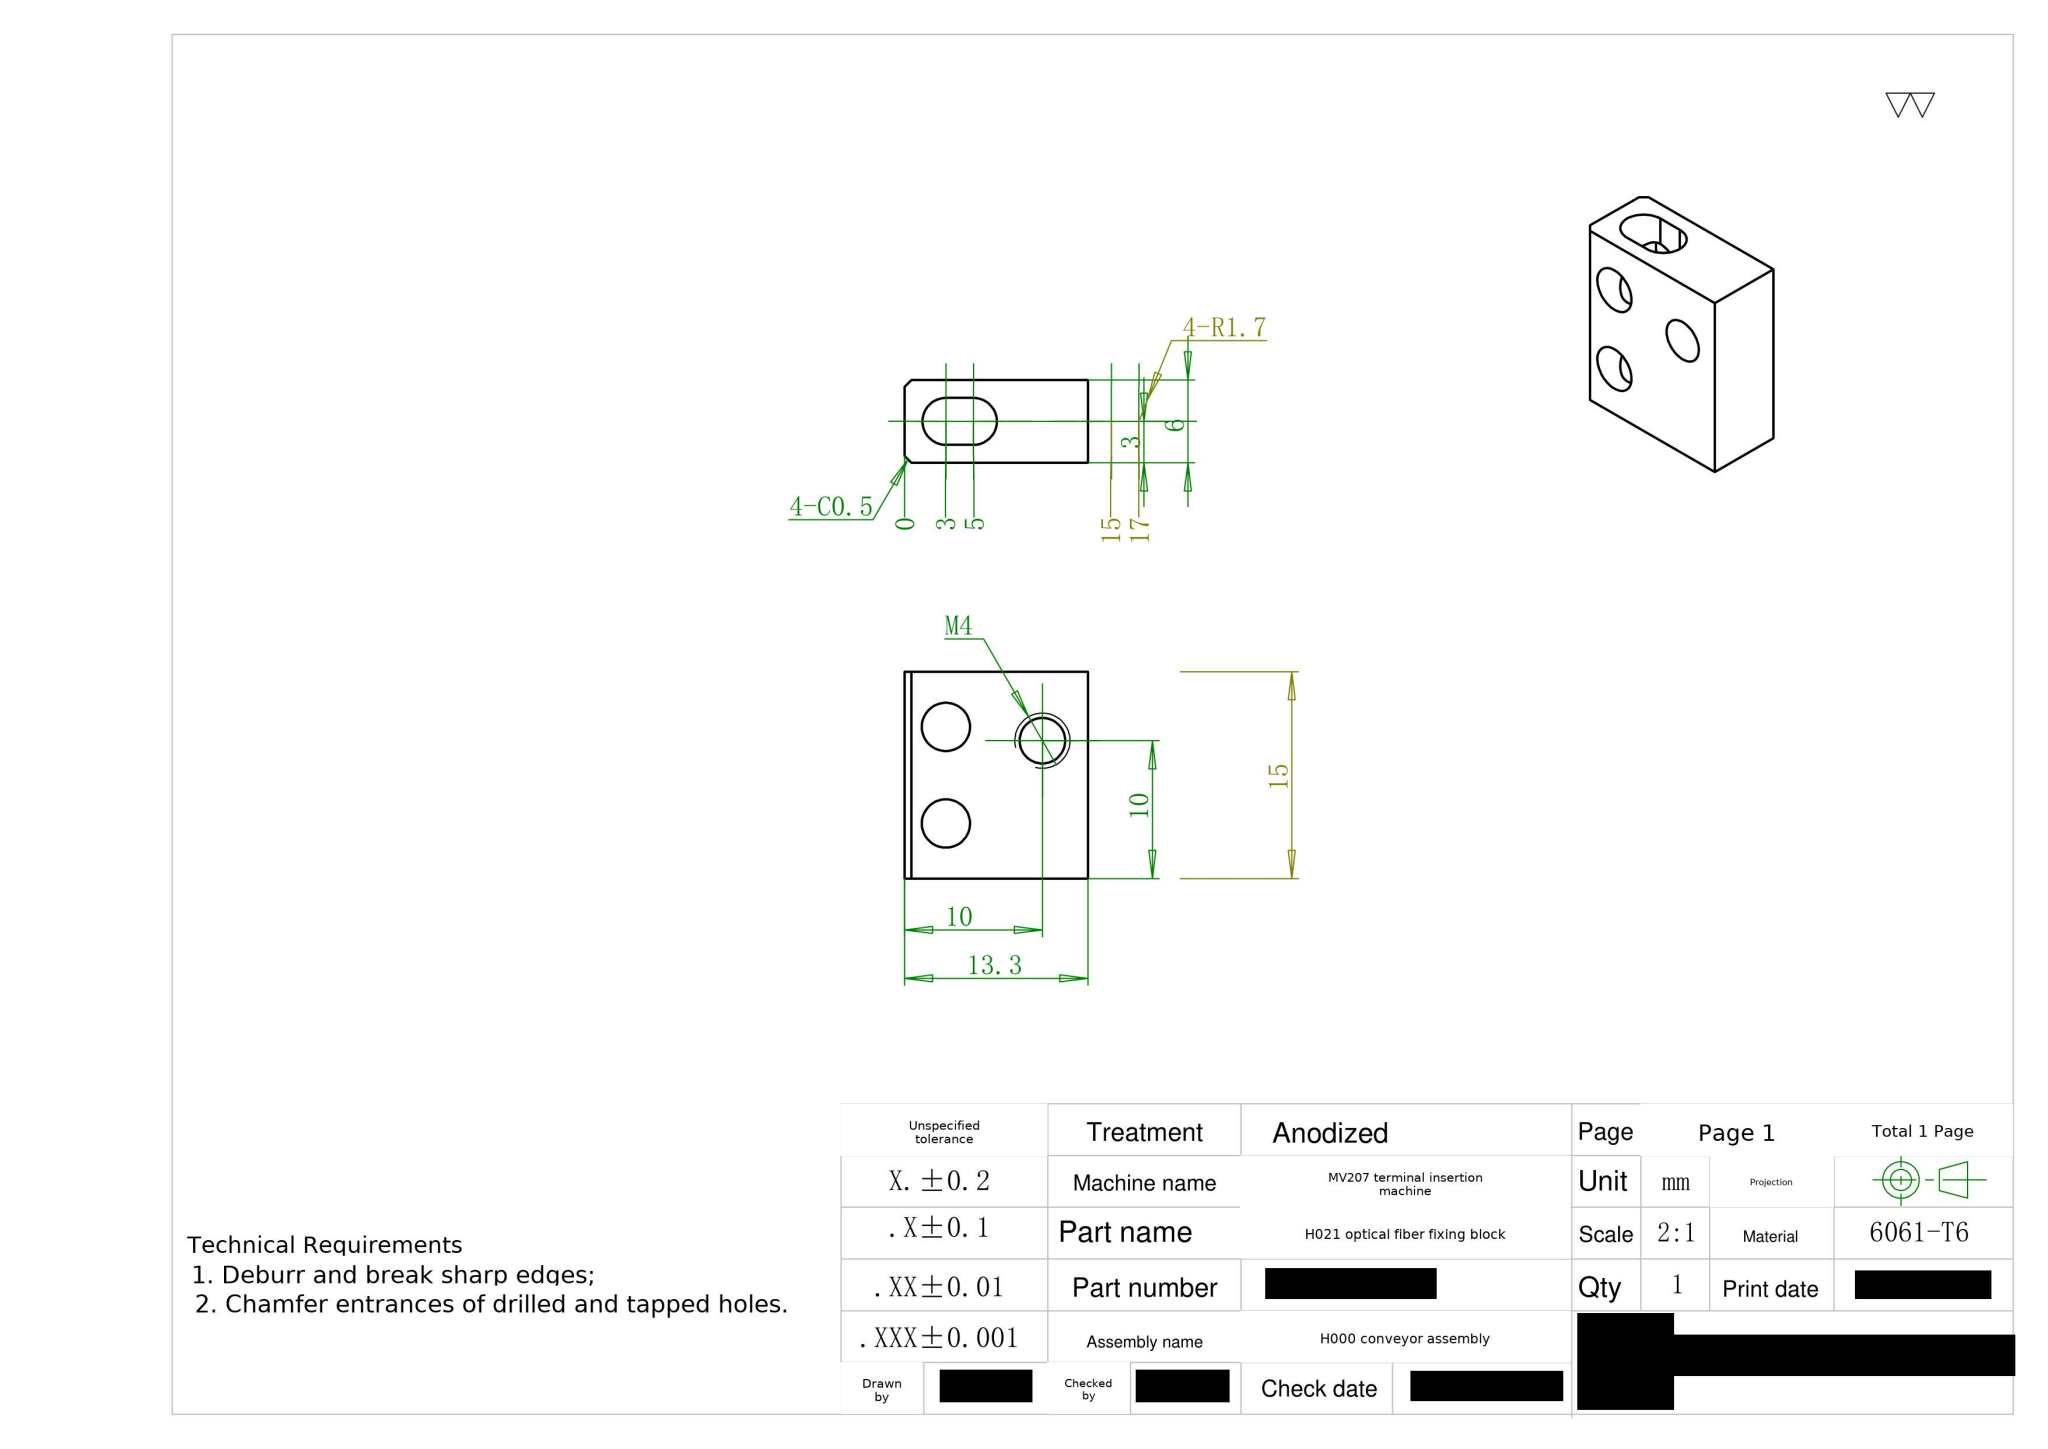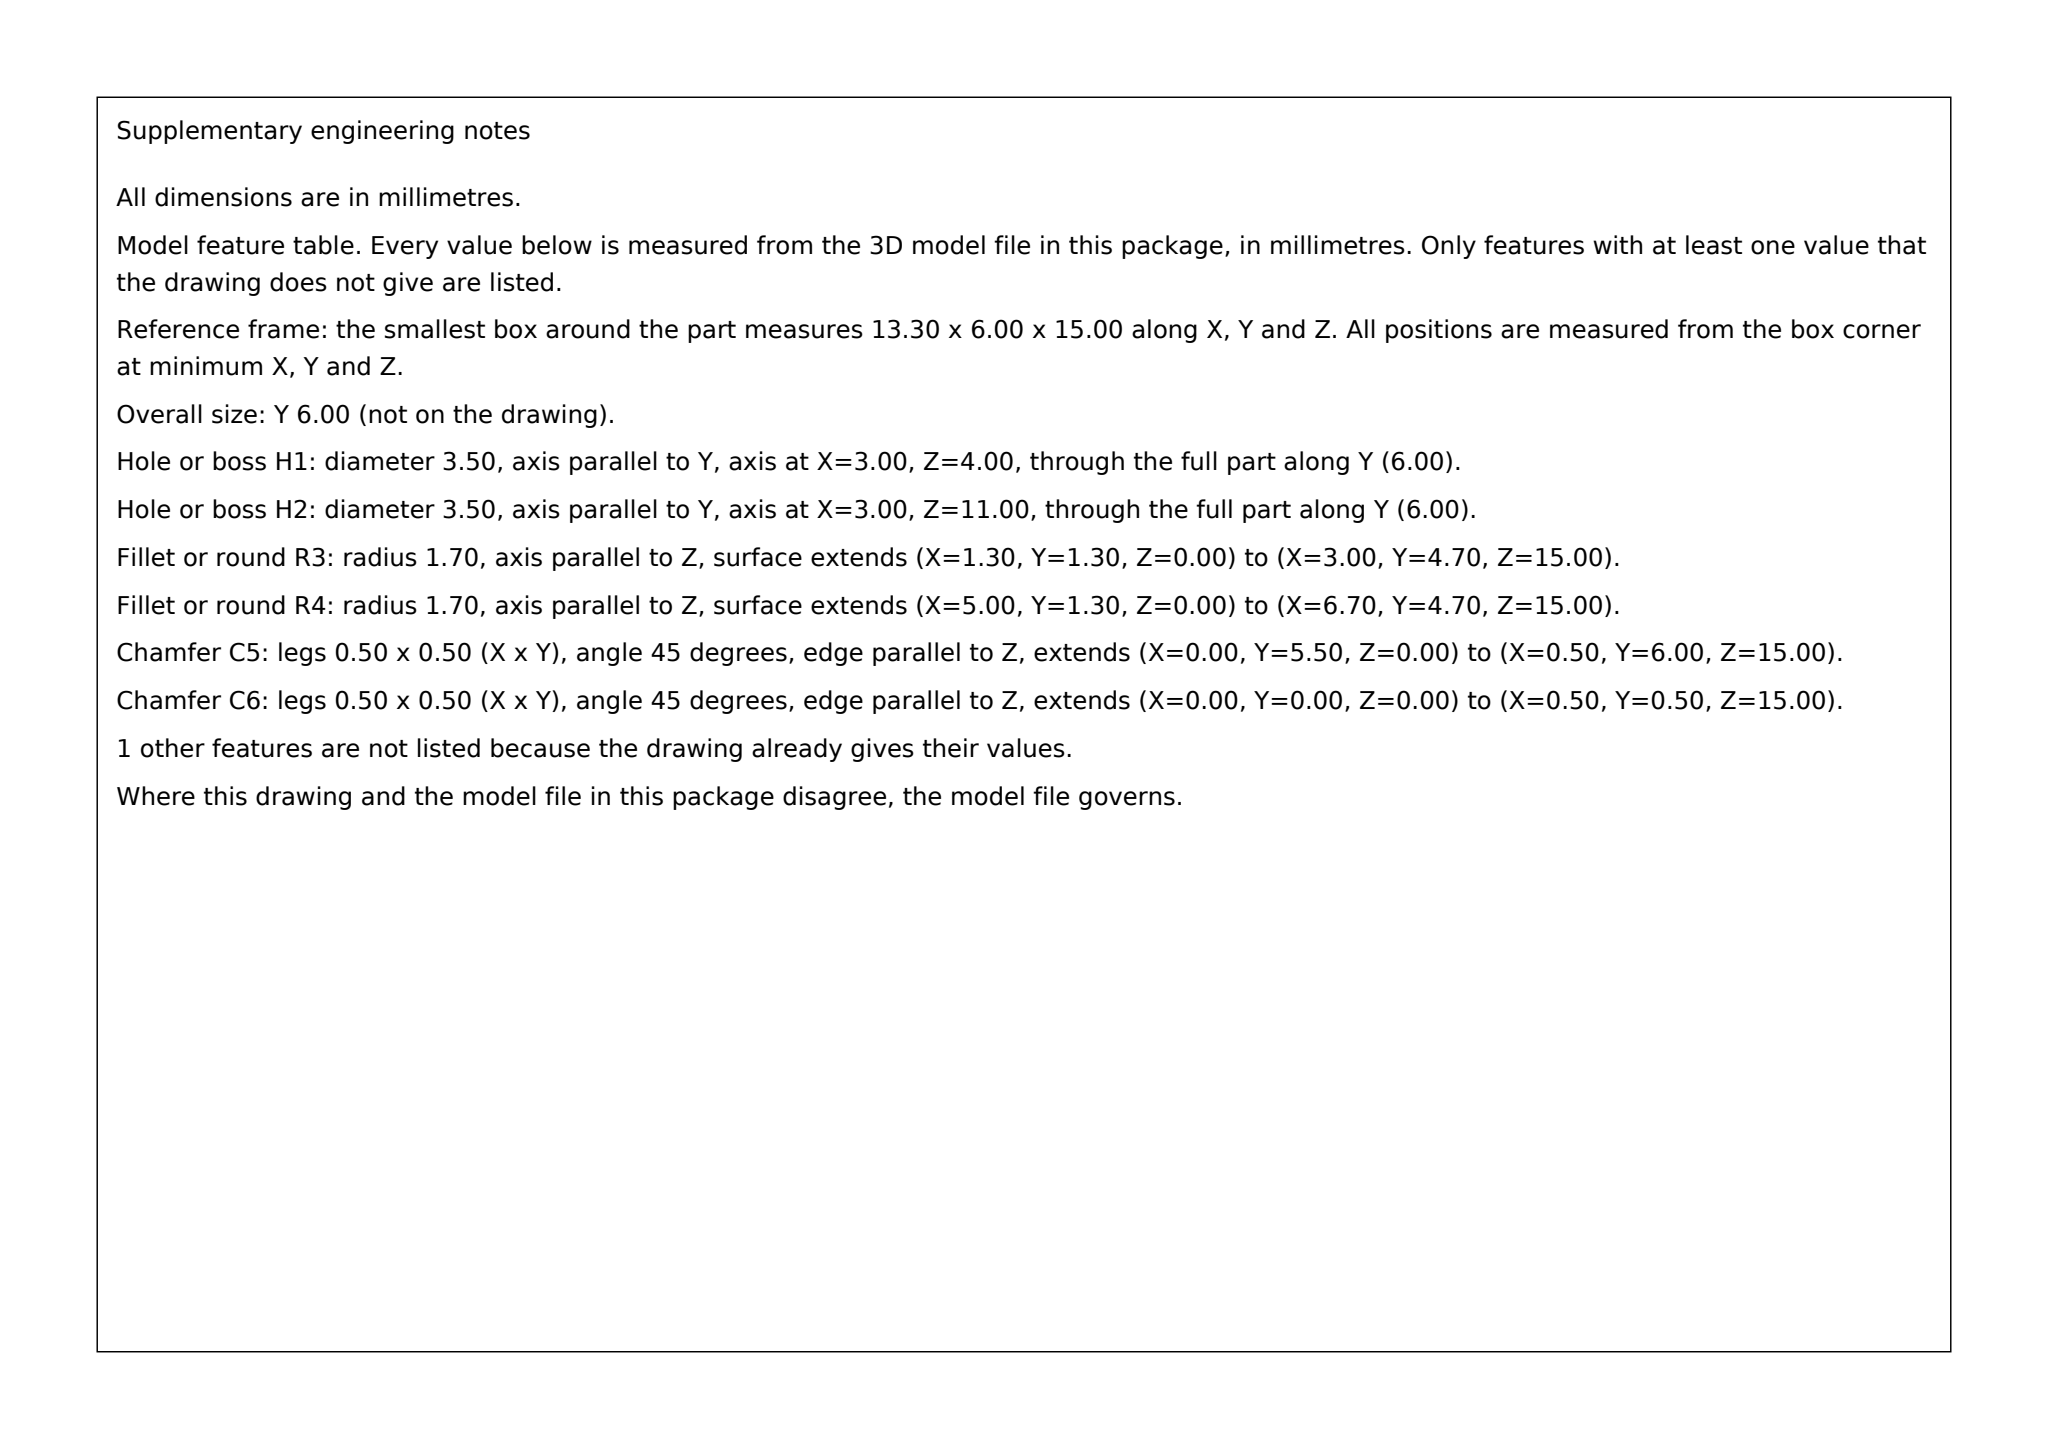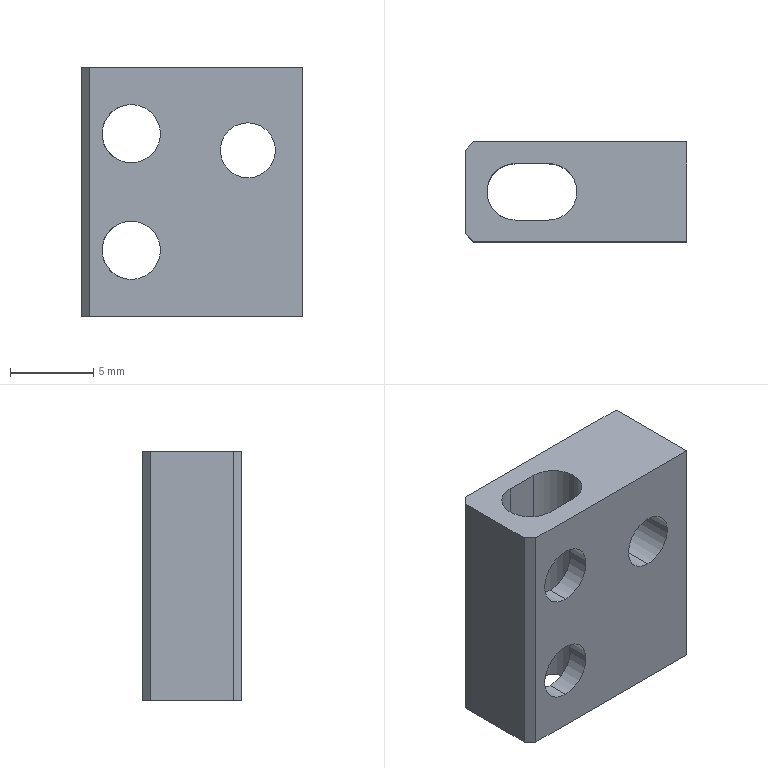Part | SolidWorks | mm | material 6061-T6 | 1 solid | 23 faces | box 13.3 x 6 x 15 mm | volume 848 mm3 | cylinder 13 | plane 10 | commonest cylinder face diameters 3.5 x6 3.4 x5 3.3 x2
build123d program:
from build123d import *

# Parameters (mm, degrees)
SKETCH1_W                  = 20
SKETCH1_H                  = 15
BOSS_EXTRUDE1_DEPTH        = 6
M4_TAPPED_HOLE1_D          = 3.3
CUT_EXTRUDE1_DEPTH         = 20
CHAMFER1_SIZE              = 0.5
F_3_5_3_5_DIAMETER_HOLE1_D = 3.5
SKETCH9_W                  = 6.7
SKETCH9_H                  = 15
CUT_EXTRUDE2_DEPTH         = 14.865


with BuildPart() as part:
    # Sketch1 → Boss-Extrude1 (new body)
    with BuildSketch(Plane(origin=(0, 0, 0), x_dir=(1, 0, 0), z_dir=(0, 1, 0))):
        Rectangle(SKETCH1_W, SKETCH1_H)
    extrude(amount=BOSS_EXTRUDE1_DEPTH)

    # M4 Tapped Hole1 (through all)
    with Locations(Plane(origin=(0, 6, 0), x_dir=(1, 0, 0), z_dir=(0, 1, 0))):
        with Locations((0, -2.5)):
            Hole(M4_TAPPED_HOLE1_D / 2)

    # Sketch4 → Cut-Extrude1 (cut, through all)
    with BuildSketch(Plane.XY.offset(7.5)):
        with BuildLine():
            Line((7, 1.3), (5, 1.3))
            ThreePointArc((5, 1.3), (3.3, 3), (5, 4.7))
            Line((5, 4.7), (7, 4.7))
            ThreePointArc((7, 4.7), (8.7, 3), (7, 1.3))
        make_face()
        with BuildLine():
            Line((-7, 1.3), (-5, 1.3))
            ThreePointArc((-5, 1.3), (-3.3, 3), (-5, 4.7))
            Line((-5, 4.7), (-7, 4.7))
            ThreePointArc((-7, 4.7), (-8.7, 3), (-7, 1.3))
        make_face()
    extrude(amount=-CUT_EXTRUDE1_DEPTH, mode=Mode.SUBTRACT)

    # Chamfer1
    chamfer1_edges = [part.edges().sort_by_distance(p)[0] for p in [
        (-10, 6, 0),
        (10, 6, 0),
        (-10, 0, 0),
        (10, 0, 0),
    ]]
    chamfer(chamfer1_edges, length=CHAMFER1_SIZE)

    # 3.5 _3.5_ Diameter Hole1 (through all)
    with Locations(Plane(origin=(0, 0, 0), x_dir=(-1, 0, 0), z_dir=(0, -1, 0))):
        with Locations((7, -3.5), (7, 3.5)):
            Hole(F_3_5_3_5_DIAMETER_HOLE1_D / 2)

    # Sketch9 → Cut-Extrude2 (cut, through all)
    with BuildSketch(Plane(origin=(0, 6, 0), x_dir=(1, 0, 0), z_dir=(0, 1, 0))):
        with Locations((6.65, 0)):
            Rectangle(SKETCH9_W, SKETCH9_H)
    extrude(amount=-CUT_EXTRUDE2_DEPTH, mode=Mode.SUBTRACT)


solid = part.part